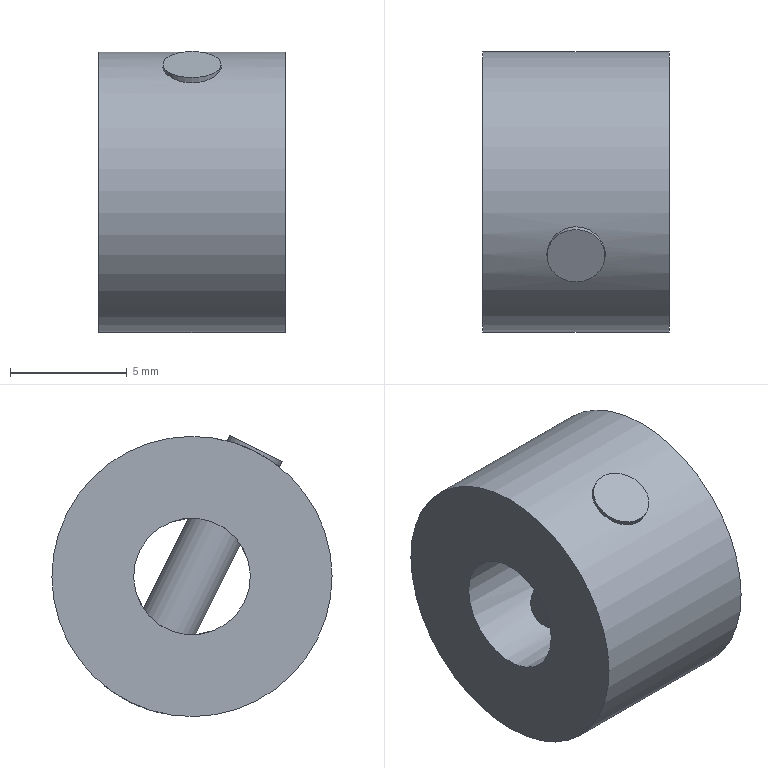Component | NX | 23E__27 | 2 solids | 9 faces | volume 772 mm3 | cylinder 5 | plane 4 | commonest cylinder face diameters 2.5 x3 12 x1 5 x1